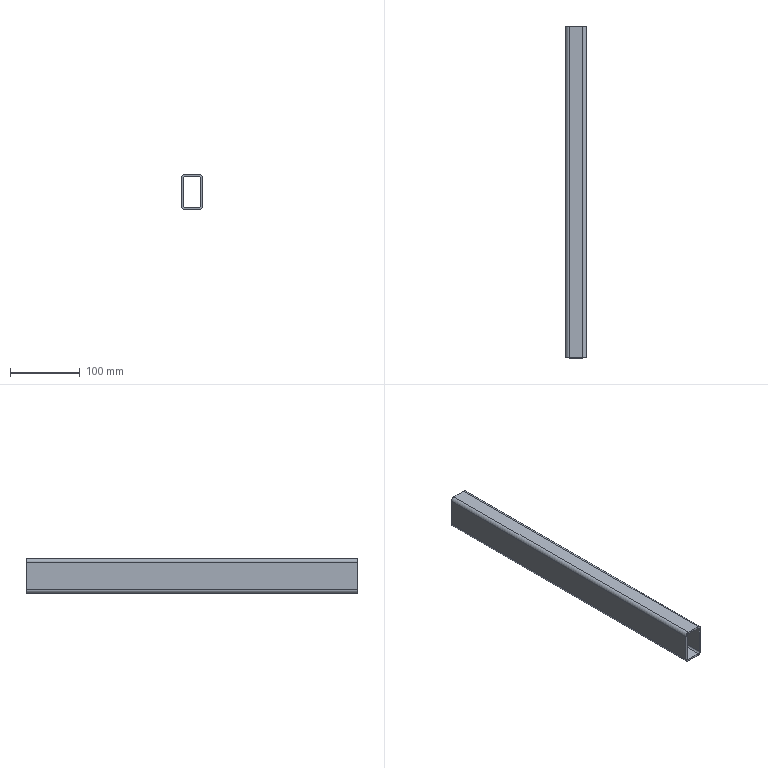Component | SolidWorks | Frame-1_SquareTube5-1 | 1 solid | 18 faces | box 30 x 475 x 50 mm | volume 176487 mm3 | plane 10 | cylinder 8 | commonest cylinder face diameters 10.4 x4 5.2 x4
STEP:
#1=COLOUR_RGB('',0.7922,0.8196,0.9333);
#2=FILL_AREA_STYLE_COLOUR('',#1);
#3=FILL_AREA_STYLE('',(#2));
#4=SURFACE_STYLE_FILL_AREA(#3);
#5=SURFACE_SIDE_STYLE('',(#4));
#6=SURFACE_STYLE_USAGE(.BOTH.,#5);
#7=PRESENTATION_STYLE_ASSIGNMENT((#6));
#8=CARTESIAN_POINT('',(20.276,-0.9843,5.717));
#9=VERTEX_POINT('',#8);
#10=CARTESIAN_POINT('',(20.276,-19.685,5.717));
#11=VERTEX_POINT('',#10);
#12=CARTESIAN_POINT('',(20.276,-19.685,5.717));
#13=DIRECTION('',(0.,-1.,0.));
#14=VECTOR('',#13,39.37);
#15=LINE('',#12,#14);
#16=EDGE_CURVE('',#9,#11,#15,.T.);
#17=ORIENTED_EDGE('',*,*,#16,.F.);
#18=CARTESIAN_POINT('',(20.276,-0.9843,7.276));
#19=VERTEX_POINT('',#18);
#20=CARTESIAN_POINT('',(20.276,-0.9843,7.276));
#21=DIRECTION('',(0.,0.,-1.));
#22=VECTOR('',#21,39.37);
#23=LINE('',#20,#22);
#24=EDGE_CURVE('',#19,#9,#23,.T.);
#25=ORIENTED_EDGE('',*,*,#24,.F.);
#26=CARTESIAN_POINT('',(20.276,-19.685,7.276));
#27=VERTEX_POINT('',#26);
#28=CARTESIAN_POINT('',(20.276,-19.685,7.276));
#29=DIRECTION('',(0.,1.,0.));
#30=VECTOR('',#29,39.37);
#31=LINE('',#28,#30);
#32=EDGE_CURVE('',#27,#19,#31,.T.);
#33=ORIENTED_EDGE('',*,*,#32,.F.);
#34=CARTESIAN_POINT('',(20.276,-19.685,7.276));
#35=DIRECTION('',(0.,0.,1.));
#36=VECTOR('',#35,39.37);
#37=LINE('',#34,#36);
#38=EDGE_CURVE('',#11,#27,#37,.T.);
#39=ORIENTED_EDGE('',*,*,#38,.F.);
#40=EDGE_LOOP('',(#17,#25,#33,#39));
#41=FACE_OUTER_BOUND('',#40,.T.);
#42=CARTESIAN_POINT('',(20.276,-19.685,7.276));
#43=DIRECTION('',(-1.,0.,0.));
#44=DIRECTION('',(0.,0.,1.));
#45=AXIS2_PLACEMENT_3D('',#42,#43,#44);
#46=PLANE('',#45);
#47=ADVANCED_FACE('',(#41),#46,.F.);
#48=CARTESIAN_POINT('',(20.071,-19.685,5.512));
#49=VERTEX_POINT('',#48);
#50=CARTESIAN_POINT('',(20.071,-19.685,5.717));
#51=DIRECTION('',(0.,-1.,0.));
#52=DIRECTION('',(0.,0.,1.));
#53=AXIS2_PLACEMENT_3D('',#50,#51,#52);
#54=CIRCLE('',#53,0.2047);
#55=EDGE_CURVE('',#49,#11,#54,.T.);
#56=ORIENTED_EDGE('',*,*,#55,.T.);
#57=ORIENTED_EDGE('',*,*,#38,.T.);
#58=CARTESIAN_POINT('',(20.071,-19.685,7.48));
#59=VERTEX_POINT('',#58);
#60=CARTESIAN_POINT('',(20.071,-19.685,7.276));
#61=DIRECTION('',(0.,-1.,0.));
#62=DIRECTION('',(0.,0.,1.));
#63=AXIS2_PLACEMENT_3D('',#60,#61,#62);
#64=CIRCLE('',#63,0.2047);
#65=EDGE_CURVE('',#27,#59,#64,.T.);
#66=ORIENTED_EDGE('',*,*,#65,.T.);
#67=CARTESIAN_POINT('',(19.299,-19.685,7.48));
#68=VERTEX_POINT('',#67);
#69=CARTESIAN_POINT('',(20.071,-19.685,7.48));
#70=DIRECTION('',(-1.,0.,0.));
#71=VECTOR('',#70,39.37);
#72=LINE('',#69,#71);
#73=EDGE_CURVE('',#59,#68,#72,.T.);
#74=ORIENTED_EDGE('',*,*,#73,.T.);
#75=CARTESIAN_POINT('',(19.094,-19.685,7.276));
#76=VERTEX_POINT('',#75);
#77=CARTESIAN_POINT('',(19.299,-19.685,7.276));
#78=DIRECTION('',(0.,-1.,0.));
#79=DIRECTION('',(0.,0.,1.));
#80=AXIS2_PLACEMENT_3D('',#77,#78,#79);
#81=CIRCLE('',#80,0.2047);
#82=EDGE_CURVE('',#68,#76,#81,.T.);
#83=ORIENTED_EDGE('',*,*,#82,.T.);
#84=CARTESIAN_POINT('',(19.094,-19.685,5.717));
#85=VERTEX_POINT('',#84);
#86=CARTESIAN_POINT('',(19.094,-19.685,7.276));
#87=DIRECTION('',(0.,-0.,-1.));
#88=VECTOR('',#87,39.37);
#89=LINE('',#86,#88);
#90=EDGE_CURVE('',#76,#85,#89,.T.);
#91=ORIENTED_EDGE('',*,*,#90,.T.);
#92=CARTESIAN_POINT('',(19.299,-19.685,5.512));
#93=VERTEX_POINT('',#92);
#94=CARTESIAN_POINT('',(19.299,-19.685,5.717));
#95=DIRECTION('',(0.,-1.,0.));
#96=DIRECTION('',(0.,0.,1.));
#97=AXIS2_PLACEMENT_3D('',#94,#95,#96);
#98=CIRCLE('',#97,0.2047);
#99=EDGE_CURVE('',#85,#93,#98,.T.);
#100=ORIENTED_EDGE('',*,*,#99,.T.);
#101=CARTESIAN_POINT('',(20.071,-19.685,5.512));
#102=DIRECTION('',(1.,0.,0.));
#103=VECTOR('',#102,39.37);
#104=LINE('',#101,#103);
#105=EDGE_CURVE('',#93,#49,#104,.T.);
#106=ORIENTED_EDGE('',*,*,#105,.T.);
#107=EDGE_LOOP('',(#56,#57,#66,#74,#83,#91,#100,#106));
#108=FACE_OUTER_BOUND('',#107,.T.);
#109=CARTESIAN_POINT('',(19.299,-19.685,5.614));
#110=VERTEX_POINT('',#109);
#111=CARTESIAN_POINT('',(19.197,-19.685,5.717));
#112=VERTEX_POINT('',#111);
#113=CARTESIAN_POINT('',(19.299,-19.685,5.717));
#114=DIRECTION('',(0.,1.,0.));
#115=DIRECTION('',(0.,0.,1.));
#116=AXIS2_PLACEMENT_3D('',#113,#114,#115);
#117=CIRCLE('',#116,0.1024);
#118=EDGE_CURVE('',#110,#112,#117,.T.);
#119=ORIENTED_EDGE('',*,*,#118,.T.);
#120=CARTESIAN_POINT('',(19.197,-19.685,7.276));
#121=VERTEX_POINT('',#120);
#122=CARTESIAN_POINT('',(19.197,-19.685,7.276));
#123=DIRECTION('',(0.,0.,1.));
#124=VECTOR('',#123,39.37);
#125=LINE('',#122,#124);
#126=EDGE_CURVE('',#112,#121,#125,.T.);
#127=ORIENTED_EDGE('',*,*,#126,.T.);
#128=CARTESIAN_POINT('',(19.299,-19.685,7.378));
#129=VERTEX_POINT('',#128);
#130=CARTESIAN_POINT('',(19.299,-19.685,7.276));
#131=DIRECTION('',(0.,1.,0.));
#132=DIRECTION('',(0.,0.,1.));
#133=AXIS2_PLACEMENT_3D('',#130,#131,#132);
#134=CIRCLE('',#133,0.1024);
#135=EDGE_CURVE('',#121,#129,#134,.T.);
#136=ORIENTED_EDGE('',*,*,#135,.T.);
#137=CARTESIAN_POINT('',(20.071,-19.685,7.378));
#138=VERTEX_POINT('',#137);
#139=CARTESIAN_POINT('',(20.071,-19.685,7.378));
#140=DIRECTION('',(1.,0.,0.));
#141=VECTOR('',#140,39.37);
#142=LINE('',#139,#141);
#143=EDGE_CURVE('',#129,#138,#142,.T.);
#144=ORIENTED_EDGE('',*,*,#143,.T.);
#145=CARTESIAN_POINT('',(20.173,-19.685,7.276));
#146=VERTEX_POINT('',#145);
#147=CARTESIAN_POINT('',(20.071,-19.685,7.276));
#148=DIRECTION('',(0.,1.,0.));
#149=DIRECTION('',(0.,0.,1.));
#150=AXIS2_PLACEMENT_3D('',#147,#148,#149);
#151=CIRCLE('',#150,0.1024);
#152=EDGE_CURVE('',#138,#146,#151,.T.);
#153=ORIENTED_EDGE('',*,*,#152,.T.);
#154=CARTESIAN_POINT('',(20.173,-19.685,5.717));
#155=VERTEX_POINT('',#154);
#156=CARTESIAN_POINT('',(20.173,-19.685,7.276));
#157=DIRECTION('',(0.,-0.,-1.));
#158=VECTOR('',#157,39.37);
#159=LINE('',#156,#158);
#160=EDGE_CURVE('',#146,#155,#159,.T.);
#161=ORIENTED_EDGE('',*,*,#160,.T.);
#162=CARTESIAN_POINT('',(20.071,-19.685,5.614));
#163=VERTEX_POINT('',#162);
#164=CARTESIAN_POINT('',(20.071,-19.685,5.717));
#165=DIRECTION('',(0.,1.,0.));
#166=DIRECTION('',(0.,0.,1.));
#167=AXIS2_PLACEMENT_3D('',#164,#165,#166);
#168=CIRCLE('',#167,0.1024);
#169=EDGE_CURVE('',#155,#163,#168,.T.);
#170=ORIENTED_EDGE('',*,*,#169,.T.);
#171=CARTESIAN_POINT('',(20.071,-19.685,5.614));
#172=DIRECTION('',(-1.,0.,0.));
#173=VECTOR('',#172,39.37);
#174=LINE('',#171,#173);
#175=EDGE_CURVE('',#163,#110,#174,.T.);
#176=ORIENTED_EDGE('',*,*,#175,.T.);
#177=EDGE_LOOP('',(#119,#127,#136,#144,#153,#161,#170,#176));
#178=FACE_BOUND('',#177,.T.);
#179=CARTESIAN_POINT('',(20.071,-19.685,7.276));
#180=DIRECTION('',(0.,-1.,0.));
#181=DIRECTION('',(0.,-0.,-1.));
#182=AXIS2_PLACEMENT_3D('',#179,#180,#181);
#183=PLANE('',#182);
#184=ADVANCED_FACE('',(#108,#178),#183,.T.);
#185=CARTESIAN_POINT('',(20.071,-0.9843,5.512));
#186=VERTEX_POINT('',#185);
#187=CARTESIAN_POINT('',(20.071,-0.9843,5.717));
#188=DIRECTION('',(0.,-1.,0.));
#189=DIRECTION('',(0.,0.,1.));
#190=AXIS2_PLACEMENT_3D('',#187,#188,#189);
#191=CIRCLE('',#190,0.2047);
#192=EDGE_CURVE('',#186,#9,#191,.T.);
#193=ORIENTED_EDGE('',*,*,#192,.T.);
#194=ORIENTED_EDGE('',*,*,#16,.T.);
#195=ORIENTED_EDGE('',*,*,#55,.F.);
#196=CARTESIAN_POINT('',(20.071,-19.685,5.512));
#197=DIRECTION('',(0.,1.,0.));
#198=VECTOR('',#197,39.37);
#199=LINE('',#196,#198);
#200=EDGE_CURVE('',#49,#186,#199,.T.);
#201=ORIENTED_EDGE('',*,*,#200,.T.);
#202=EDGE_LOOP('',(#193,#194,#195,#201));
#203=FACE_OUTER_BOUND('',#202,.T.);
#204=CARTESIAN_POINT('',(20.071,-19.685,5.717));
#205=DIRECTION('',(0.,1.,0.));
#206=DIRECTION('',(0.,0.,1.));
#207=AXIS2_PLACEMENT_3D('',#204,#205,#206);
#208=CYLINDRICAL_SURFACE('',#207,0.2047);
#209=ADVANCED_FACE('',(#203),#208,.T.);
#210=ORIENTED_EDGE('',*,*,#192,.F.);
#211=CARTESIAN_POINT('',(19.299,-0.9843,5.512));
#212=VERTEX_POINT('',#211);
#213=CARTESIAN_POINT('',(-19.492,-0.9843,5.512));
#214=DIRECTION('',(1.,0.,0.));
#215=VECTOR('',#214,39.37);
#216=LINE('',#213,#215);
#217=EDGE_CURVE('',#212,#186,#216,.T.);
#218=ORIENTED_EDGE('',*,*,#217,.F.);
#219=CARTESIAN_POINT('',(19.094,-0.9843,5.717));
#220=VERTEX_POINT('',#219);
#221=CARTESIAN_POINT('',(19.299,-0.9843,5.717));
#222=DIRECTION('',(0.,-1.,0.));
#223=DIRECTION('',(0.,0.,1.));
#224=AXIS2_PLACEMENT_3D('',#221,#222,#223);
#225=CIRCLE('',#224,0.2047);
#226=EDGE_CURVE('',#220,#212,#225,.T.);
#227=ORIENTED_EDGE('',*,*,#226,.F.);
#228=CARTESIAN_POINT('',(19.094,-0.9843,7.276));
#229=VERTEX_POINT('',#228);
#230=CARTESIAN_POINT('',(19.094,-0.9843,7.083));
#231=DIRECTION('',(0.,0.,-1.));
#232=VECTOR('',#231,39.37);
#233=LINE('',#230,#232);
#234=EDGE_CURVE('',#229,#220,#233,.T.);
#235=ORIENTED_EDGE('',*,*,#234,.F.);
#236=CARTESIAN_POINT('',(19.299,-0.9843,7.48));
#237=VERTEX_POINT('',#236);
#238=CARTESIAN_POINT('',(19.299,-0.9843,7.276));
#239=DIRECTION('',(0.,-1.,0.));
#240=DIRECTION('',(0.,0.,1.));
#241=AXIS2_PLACEMENT_3D('',#238,#239,#240);
#242=CIRCLE('',#241,0.2047);
#243=EDGE_CURVE('',#237,#229,#242,.T.);
#244=ORIENTED_EDGE('',*,*,#243,.F.);
#245=CARTESIAN_POINT('',(20.071,-0.9843,7.48));
#246=VERTEX_POINT('',#245);
#247=CARTESIAN_POINT('',(-19.492,-0.9843,7.48));
#248=DIRECTION('',(-1.,0.,0.));
#249=VECTOR('',#248,39.37);
#250=LINE('',#247,#249);
#251=EDGE_CURVE('',#246,#237,#250,.T.);
#252=ORIENTED_EDGE('',*,*,#251,.F.);
#253=CARTESIAN_POINT('',(20.071,-0.9843,7.276));
#254=DIRECTION('',(0.,-1.,0.));
#255=DIRECTION('',(0.,0.,1.));
#256=AXIS2_PLACEMENT_3D('',#253,#254,#255);
#257=CIRCLE('',#256,0.2047);
#258=EDGE_CURVE('',#19,#246,#257,.T.);
#259=ORIENTED_EDGE('',*,*,#258,.F.);
#260=ORIENTED_EDGE('',*,*,#24,.T.);
#261=EDGE_LOOP('',(#210,#218,#227,#235,#244,#252,#259,#260));
#262=FACE_OUTER_BOUND('',#261,.T.);
#263=CARTESIAN_POINT('',(19.197,-0.9843,5.717));
#264=VERTEX_POINT('',#263);
#265=CARTESIAN_POINT('',(19.197,-0.9843,7.276));
#266=VERTEX_POINT('',#265);
#267=CARTESIAN_POINT('',(19.197,-0.9843,7.083));
#268=DIRECTION('',(0.,0.,1.));
#269=VECTOR('',#268,39.37);
#270=LINE('',#267,#269);
#271=EDGE_CURVE('',#264,#266,#270,.T.);
#272=ORIENTED_EDGE('',*,*,#271,.F.);
#273=CARTESIAN_POINT('',(19.299,-0.9843,5.614));
#274=VERTEX_POINT('',#273);
#275=CARTESIAN_POINT('',(19.299,-0.9843,5.717));
#276=DIRECTION('',(0.,1.,0.));
#277=DIRECTION('',(0.,0.,1.));
#278=AXIS2_PLACEMENT_3D('',#275,#276,#277);
#279=CIRCLE('',#278,0.1024);
#280=EDGE_CURVE('',#274,#264,#279,.T.);
#281=ORIENTED_EDGE('',*,*,#280,.F.);
#282=CARTESIAN_POINT('',(20.071,-0.9843,5.614));
#283=VERTEX_POINT('',#282);
#284=CARTESIAN_POINT('',(-19.492,-0.9843,5.614));
#285=DIRECTION('',(-1.,0.,0.));
#286=VECTOR('',#285,39.37);
#287=LINE('',#284,#286);
#288=EDGE_CURVE('',#283,#274,#287,.T.);
#289=ORIENTED_EDGE('',*,*,#288,.F.);
#290=CARTESIAN_POINT('',(20.173,-0.9843,5.717));
#291=VERTEX_POINT('',#290);
#292=CARTESIAN_POINT('',(20.071,-0.9843,5.717));
#293=DIRECTION('',(0.,1.,0.));
#294=DIRECTION('',(0.,0.,1.));
#295=AXIS2_PLACEMENT_3D('',#292,#293,#294);
#296=CIRCLE('',#295,0.1024);
#297=EDGE_CURVE('',#291,#283,#296,.T.);
#298=ORIENTED_EDGE('',*,*,#297,.F.);
#299=CARTESIAN_POINT('',(20.173,-0.9843,7.276));
#300=VERTEX_POINT('',#299);
#301=CARTESIAN_POINT('',(20.173,-0.9843,7.083));
#302=DIRECTION('',(0.,0.,-1.));
#303=VECTOR('',#302,39.37);
#304=LINE('',#301,#303);
#305=EDGE_CURVE('',#300,#291,#304,.T.);
#306=ORIENTED_EDGE('',*,*,#305,.F.);
#307=CARTESIAN_POINT('',(20.071,-0.9843,7.378));
#308=VERTEX_POINT('',#307);
#309=CARTESIAN_POINT('',(20.071,-0.9843,7.276));
#310=DIRECTION('',(0.,1.,0.));
#311=DIRECTION('',(0.,0.,1.));
#312=AXIS2_PLACEMENT_3D('',#309,#310,#311);
#313=CIRCLE('',#312,0.1024);
#314=EDGE_CURVE('',#308,#300,#313,.T.);
#315=ORIENTED_EDGE('',*,*,#314,.F.);
#316=CARTESIAN_POINT('',(19.299,-0.9843,7.378));
#317=VERTEX_POINT('',#316);
#318=CARTESIAN_POINT('',(-19.492,-0.9843,7.378));
#319=DIRECTION('',(1.,0.,0.));
#320=VECTOR('',#319,39.37);
#321=LINE('',#318,#320);
#322=EDGE_CURVE('',#317,#308,#321,.T.);
#323=ORIENTED_EDGE('',*,*,#322,.F.);
#324=CARTESIAN_POINT('',(19.299,-0.9843,7.276));
#325=DIRECTION('',(0.,1.,0.));
#326=DIRECTION('',(0.,0.,1.));
#327=AXIS2_PLACEMENT_3D('',#324,#325,#326);
#328=CIRCLE('',#327,0.1024);
#329=EDGE_CURVE('',#266,#317,#328,.T.);
#330=ORIENTED_EDGE('',*,*,#329,.F.);
#331=EDGE_LOOP('',(#272,#281,#289,#298,#306,#315,#323,#330));
#332=FACE_BOUND('',#331,.T.);
#333=CARTESIAN_POINT('',(-19.492,-0.9843,7.083));
#334=DIRECTION('',(0.,-1.,0.));
#335=DIRECTION('',(0.,0.,-1.));
#336=AXIS2_PLACEMENT_3D('',#333,#334,#335);
#337=PLANE('',#336);
#338=ADVANCED_FACE('',(#262,#332),#337,.F.);
#339=ORIENTED_EDGE('',*,*,#258,.T.);
#340=CARTESIAN_POINT('',(20.071,-19.685,7.48));
#341=DIRECTION('',(0.,-1.,0.));
#342=VECTOR('',#341,39.37);
#343=LINE('',#340,#342);
#344=EDGE_CURVE('',#246,#59,#343,.T.);
#345=ORIENTED_EDGE('',*,*,#344,.T.);
#346=ORIENTED_EDGE('',*,*,#65,.F.);
#347=ORIENTED_EDGE('',*,*,#32,.T.);
#348=EDGE_LOOP('',(#339,#345,#346,#347));
#349=FACE_OUTER_BOUND('',#348,.T.);
#350=CARTESIAN_POINT('',(20.071,-19.685,7.276));
#351=DIRECTION('',(0.,1.,0.));
#352=DIRECTION('',(0.,0.,1.));
#353=AXIS2_PLACEMENT_3D('',#350,#351,#352);
#354=CYLINDRICAL_SURFACE('',#353,0.2047);
#355=ADVANCED_FACE('',(#349),#354,.T.);
#356=CARTESIAN_POINT('',(19.299,-19.685,5.512));
#357=DIRECTION('',(0.,-1.,0.));
#358=VECTOR('',#357,39.37);
#359=LINE('',#356,#358);
#360=EDGE_CURVE('',#212,#93,#359,.T.);
#361=ORIENTED_EDGE('',*,*,#360,.F.);
#362=ORIENTED_EDGE('',*,*,#217,.T.);
#363=ORIENTED_EDGE('',*,*,#200,.F.);
#364=ORIENTED_EDGE('',*,*,#105,.F.);
#365=EDGE_LOOP('',(#361,#362,#363,#364));
#366=FACE_OUTER_BOUND('',#365,.T.);
#367=CARTESIAN_POINT('',(19.299,-19.685,5.512));
#368=DIRECTION('',(0.,0.,1.));
#369=DIRECTION('',(1.,0.,0.));
#370=AXIS2_PLACEMENT_3D('',#367,#368,#369);
#371=PLANE('',#370);
#372=ADVANCED_FACE('',(#366),#371,.F.);
#373=ORIENTED_EDGE('',*,*,#226,.T.);
#374=ORIENTED_EDGE('',*,*,#360,.T.);
#375=ORIENTED_EDGE('',*,*,#99,.F.);
#376=CARTESIAN_POINT('',(19.094,-19.685,5.717));
#377=DIRECTION('',(0.,1.,0.));
#378=VECTOR('',#377,39.37);
#379=LINE('',#376,#378);
#380=EDGE_CURVE('',#85,#220,#379,.T.);
#381=ORIENTED_EDGE('',*,*,#380,.T.);
#382=EDGE_LOOP('',(#373,#374,#375,#381));
#383=FACE_OUTER_BOUND('',#382,.T.);
#384=CARTESIAN_POINT('',(19.299,-19.685,5.717));
#385=DIRECTION('',(0.,1.,0.));
#386=DIRECTION('',(0.,0.,1.));
#387=AXIS2_PLACEMENT_3D('',#384,#385,#386);
#388=CYLINDRICAL_SURFACE('',#387,0.2047);
#389=ADVANCED_FACE('',(#383),#388,.T.);
#390=CARTESIAN_POINT('',(19.094,-19.685,7.276));
#391=DIRECTION('',(0.,-1.,0.));
#392=VECTOR('',#391,39.37);
#393=LINE('',#390,#392);
#394=EDGE_CURVE('',#229,#76,#393,.T.);
#395=ORIENTED_EDGE('',*,*,#394,.F.);
#396=ORIENTED_EDGE('',*,*,#234,.T.);
#397=ORIENTED_EDGE('',*,*,#380,.F.);
#398=ORIENTED_EDGE('',*,*,#90,.F.);
#399=EDGE_LOOP('',(#395,#396,#397,#398));
#400=FACE_OUTER_BOUND('',#399,.T.);
#401=CARTESIAN_POINT('',(19.094,-19.685,5.717));
#402=DIRECTION('',(1.,0.,0.));
#403=DIRECTION('',(0.,0.,-1.));
#404=AXIS2_PLACEMENT_3D('',#401,#402,#403);
#405=PLANE('',#404);
#406=ADVANCED_FACE('',(#400),#405,.F.);
#407=ORIENTED_EDGE('',*,*,#243,.T.);
#408=ORIENTED_EDGE('',*,*,#394,.T.);
#409=ORIENTED_EDGE('',*,*,#82,.F.);
#410=CARTESIAN_POINT('',(19.299,-19.685,7.48));
#411=DIRECTION('',(0.,1.,0.));
#412=VECTOR('',#411,39.37);
#413=LINE('',#410,#412);
#414=EDGE_CURVE('',#68,#237,#413,.T.);
#415=ORIENTED_EDGE('',*,*,#414,.T.);
#416=EDGE_LOOP('',(#407,#408,#409,#415));
#417=FACE_OUTER_BOUND('',#416,.T.);
#418=CARTESIAN_POINT('',(19.299,-19.685,7.276));
#419=DIRECTION('',(0.,1.,0.));
#420=DIRECTION('',(0.,0.,1.));
#421=AXIS2_PLACEMENT_3D('',#418,#419,#420);
#422=CYLINDRICAL_SURFACE('',#421,0.2047);
#423=ADVANCED_FACE('',(#417),#422,.T.);
#424=ORIENTED_EDGE('',*,*,#344,.F.);
#425=ORIENTED_EDGE('',*,*,#251,.T.);
#426=ORIENTED_EDGE('',*,*,#414,.F.);
#427=ORIENTED_EDGE('',*,*,#73,.F.);
#428=EDGE_LOOP('',(#424,#425,#426,#427));
#429=FACE_OUTER_BOUND('',#428,.T.);
#430=CARTESIAN_POINT('',(20.071,-19.685,7.48));
#431=DIRECTION('',(0.,0.,-1.));
#432=DIRECTION('',(-1.,0.,0.));
#433=AXIS2_PLACEMENT_3D('',#430,#431,#432);
#434=PLANE('',#433);
#435=ADVANCED_FACE('',(#429),#434,.F.);
#436=CARTESIAN_POINT('',(19.197,-19.685,5.717));
#437=DIRECTION('',(0.,1.,0.));
#438=VECTOR('',#437,39.37);
#439=LINE('',#436,#438);
#440=EDGE_CURVE('',#112,#264,#439,.T.);
#441=ORIENTED_EDGE('',*,*,#440,.T.);
#442=ORIENTED_EDGE('',*,*,#271,.T.);
#443=CARTESIAN_POINT('',(19.197,-19.685,7.276));
#444=DIRECTION('',(0.,-1.,0.));
#445=VECTOR('',#444,39.37);
#446=LINE('',#443,#445);
#447=EDGE_CURVE('',#266,#121,#446,.T.);
#448=ORIENTED_EDGE('',*,*,#447,.T.);
#449=ORIENTED_EDGE('',*,*,#126,.F.);
#450=EDGE_LOOP('',(#441,#442,#448,#449));
#451=FACE_OUTER_BOUND('',#450,.T.);
#452=CARTESIAN_POINT('',(19.197,-19.685,5.717));
#453=DIRECTION('',(1.,0.,0.));
#454=DIRECTION('',(0.,0.,-1.));
#455=AXIS2_PLACEMENT_3D('',#452,#453,#454);
#456=PLANE('',#455);
#457=ADVANCED_FACE('',(#451),#456,.T.);
#458=ORIENTED_EDGE('',*,*,#118,.F.);
#459=CARTESIAN_POINT('',(19.299,-19.685,5.614));
#460=DIRECTION('',(0.,-1.,0.));
#461=VECTOR('',#460,39.37);
#462=LINE('',#459,#461);
#463=EDGE_CURVE('',#274,#110,#462,.T.);
#464=ORIENTED_EDGE('',*,*,#463,.F.);
#465=ORIENTED_EDGE('',*,*,#280,.T.);
#466=ORIENTED_EDGE('',*,*,#440,.F.);
#467=EDGE_LOOP('',(#458,#464,#465,#466));
#468=FACE_OUTER_BOUND('',#467,.T.);
#469=CARTESIAN_POINT('',(19.299,-19.685,5.717));
#470=DIRECTION('',(0.,1.,0.));
#471=DIRECTION('',(0.,0.,1.));
#472=AXIS2_PLACEMENT_3D('',#469,#470,#471);
#473=CYLINDRICAL_SURFACE('',#472,0.1024);
#474=ADVANCED_FACE('',(#468),#473,.F.);
#475=CARTESIAN_POINT('',(20.071,-19.685,5.614));
#476=DIRECTION('',(0.,1.,0.));
#477=VECTOR('',#476,39.37);
#478=LINE('',#475,#477);
#479=EDGE_CURVE('',#163,#283,#478,.T.);
#480=ORIENTED_EDGE('',*,*,#479,.T.);
#481=ORIENTED_EDGE('',*,*,#288,.T.);
#482=ORIENTED_EDGE('',*,*,#463,.T.);
#483=ORIENTED_EDGE('',*,*,#175,.F.);
#484=EDGE_LOOP('',(#480,#481,#482,#483));
#485=FACE_OUTER_BOUND('',#484,.T.);
#486=CARTESIAN_POINT('',(19.299,-19.685,5.614));
#487=DIRECTION('',(0.,0.,1.));
#488=DIRECTION('',(1.,0.,0.));
#489=AXIS2_PLACEMENT_3D('',#486,#487,#488);
#490=PLANE('',#489);
#491=ADVANCED_FACE('',(#485),#490,.T.);
#492=ORIENTED_EDGE('',*,*,#169,.F.);
#493=CARTESIAN_POINT('',(20.173,-19.685,5.717));
#494=DIRECTION('',(0.,-1.,0.));
#495=VECTOR('',#494,39.37);
#496=LINE('',#493,#495);
#497=EDGE_CURVE('',#291,#155,#496,.T.);
#498=ORIENTED_EDGE('',*,*,#497,.F.);
#499=ORIENTED_EDGE('',*,*,#297,.T.);
#500=ORIENTED_EDGE('',*,*,#479,.F.);
#501=EDGE_LOOP('',(#492,#498,#499,#500));
#502=FACE_OUTER_BOUND('',#501,.T.);
#503=CARTESIAN_POINT('',(20.071,-19.685,5.717));
#504=DIRECTION('',(0.,1.,0.));
#505=DIRECTION('',(0.,0.,1.));
#506=AXIS2_PLACEMENT_3D('',#503,#504,#505);
#507=CYLINDRICAL_SURFACE('',#506,0.1024);
#508=ADVANCED_FACE('',(#502),#507,.F.);
#509=CARTESIAN_POINT('',(20.173,-19.685,7.276));
#510=DIRECTION('',(0.,1.,0.));
#511=VECTOR('',#510,39.37);
#512=LINE('',#509,#511);
#513=EDGE_CURVE('',#146,#300,#512,.T.);
#514=ORIENTED_EDGE('',*,*,#513,.T.);
#515=ORIENTED_EDGE('',*,*,#305,.T.);
#516=ORIENTED_EDGE('',*,*,#497,.T.);
#517=ORIENTED_EDGE('',*,*,#160,.F.);
#518=EDGE_LOOP('',(#514,#515,#516,#517));
#519=FACE_OUTER_BOUND('',#518,.T.);
#520=CARTESIAN_POINT('',(20.173,-19.685,7.276));
#521=DIRECTION('',(-1.,0.,0.));
#522=DIRECTION('',(0.,0.,1.));
#523=AXIS2_PLACEMENT_3D('',#520,#521,#522);
#524=PLANE('',#523);
#525=ADVANCED_FACE('',(#519),#524,.T.);
#526=ORIENTED_EDGE('',*,*,#152,.F.);
#527=CARTESIAN_POINT('',(20.071,-19.685,7.378));
#528=DIRECTION('',(0.,-1.,0.));
#529=VECTOR('',#528,39.37);
#530=LINE('',#527,#529);
#531=EDGE_CURVE('',#308,#138,#530,.T.);
#532=ORIENTED_EDGE('',*,*,#531,.F.);
#533=ORIENTED_EDGE('',*,*,#314,.T.);
#534=ORIENTED_EDGE('',*,*,#513,.F.);
#535=EDGE_LOOP('',(#526,#532,#533,#534));
#536=FACE_OUTER_BOUND('',#535,.T.);
#537=CARTESIAN_POINT('',(20.071,-19.685,7.276));
#538=DIRECTION('',(0.,1.,0.));
#539=DIRECTION('',(0.,0.,1.));
#540=AXIS2_PLACEMENT_3D('',#537,#538,#539);
#541=CYLINDRICAL_SURFACE('',#540,0.1024);
#542=ADVANCED_FACE('',(#536),#541,.F.);
#543=CARTESIAN_POINT('',(19.299,-19.685,7.378));
#544=DIRECTION('',(0.,1.,0.));
#545=VECTOR('',#544,39.37);
#546=LINE('',#543,#545);
#547=EDGE_CURVE('',#129,#317,#546,.T.);
#548=ORIENTED_EDGE('',*,*,#547,.T.);
#549=ORIENTED_EDGE('',*,*,#322,.T.);
#550=ORIENTED_EDGE('',*,*,#531,.T.);
#551=ORIENTED_EDGE('',*,*,#143,.F.);
#552=EDGE_LOOP('',(#548,#549,#550,#551));
#553=FACE_OUTER_BOUND('',#552,.T.);
#554=CARTESIAN_POINT('',(20.071,-19.685,7.378));
#555=DIRECTION('',(0.,0.,-1.));
#556=DIRECTION('',(-1.,0.,0.));
#557=AXIS2_PLACEMENT_3D('',#554,#555,#556);
#558=PLANE('',#557);
#559=ADVANCED_FACE('',(#553),#558,.T.);
#560=ORIENTED_EDGE('',*,*,#135,.F.);
#561=ORIENTED_EDGE('',*,*,#447,.F.);
#562=ORIENTED_EDGE('',*,*,#329,.T.);
#563=ORIENTED_EDGE('',*,*,#547,.F.);
#564=EDGE_LOOP('',(#560,#561,#562,#563));
#565=FACE_OUTER_BOUND('',#564,.T.);
#566=CARTESIAN_POINT('',(19.299,-19.685,7.276));
#567=DIRECTION('',(0.,1.,0.));
#568=DIRECTION('',(0.,0.,1.));
#569=AXIS2_PLACEMENT_3D('',#566,#567,#568);
#570=CYLINDRICAL_SURFACE('',#569,0.1024);
#571=ADVANCED_FACE('',(#565),#570,.F.);
#572=CLOSED_SHELL('',(#47,#184,#209,#338,#355,#372,#389,#406,#423,#435,#457,#474,#491,#508,#525,#542,#559,#571));
#573=MANIFOLD_SOLID_BREP('',#572);
#574=STYLED_ITEM('',(#7),#573);
#575=(LENGTH_UNIT()NAMED_UNIT(*)SI_UNIT($,.METRE.));
#576=LENGTH_MEASURE_WITH_UNIT(LENGTH_MEASURE(0.0254),#575);
#577=DIMENSIONAL_EXPONENTS(1.,0.,0.,0.,0.,0.,0.);
#578=(CONVERSION_BASED_UNIT('',#576)LENGTH_UNIT()NAMED_UNIT(#577));
#579=UNCERTAINTY_MEASURE_WITH_UNIT(LENGTH_MEASURE(0.00001),#578,'','');
#580=(NAMED_UNIT(*)PLANE_ANGLE_UNIT()SI_UNIT($,.RADIAN.));
#581=(NAMED_UNIT(*)SI_UNIT($,.STERADIAN.)SOLID_ANGLE_UNIT());
#582=(GEOMETRIC_REPRESENTATION_CONTEXT(3)GLOBAL_UNCERTAINTY_ASSIGNED_CONTEXT((#579))GLOBAL_UNIT_ASSIGNED_CONTEXT((#578,#580,#581))REPRESENTATION_CONTEXT('',''));
#583=MECHANICAL_DESIGN_GEOMETRIC_PRESENTATION_REPRESENTATION('',(#574),#582);
#584=CARTESIAN_POINT('',(0.,0.,0.));
#585=DIRECTION('',(0.,0.,1.));
#586=DIRECTION('',(1.,0.,0.));
#587=AXIS2_PLACEMENT_3D('',#584,#585,#586);
#588=(LENGTH_UNIT()NAMED_UNIT(*)SI_UNIT($,.METRE.));
#589=LENGTH_MEASURE_WITH_UNIT(LENGTH_MEASURE(0.0254),#588);
#590=DIMENSIONAL_EXPONENTS(1.,0.,0.,0.,0.,0.,0.);
#591=(CONVERSION_BASED_UNIT('',#589)LENGTH_UNIT()NAMED_UNIT(#590));
#592=UNCERTAINTY_MEASURE_WITH_UNIT(LENGTH_MEASURE(0.00001),#591,'','');
#593=(NAMED_UNIT(*)PLANE_ANGLE_UNIT()SI_UNIT($,.RADIAN.));
#594=(NAMED_UNIT(*)SI_UNIT($,.STERADIAN.)SOLID_ANGLE_UNIT());
#595=(GEOMETRIC_REPRESENTATION_CONTEXT(3)GLOBAL_UNCERTAINTY_ASSIGNED_CONTEXT((#592))GLOBAL_UNIT_ASSIGNED_CONTEXT((#591,#593,#594))REPRESENTATION_CONTEXT('',''));
#596=ADVANCED_BREP_SHAPE_REPRESENTATION('',(#573,#587),#595);
#597=PRESENTATION_LAYER_ASSIGNMENT('','',(#574));